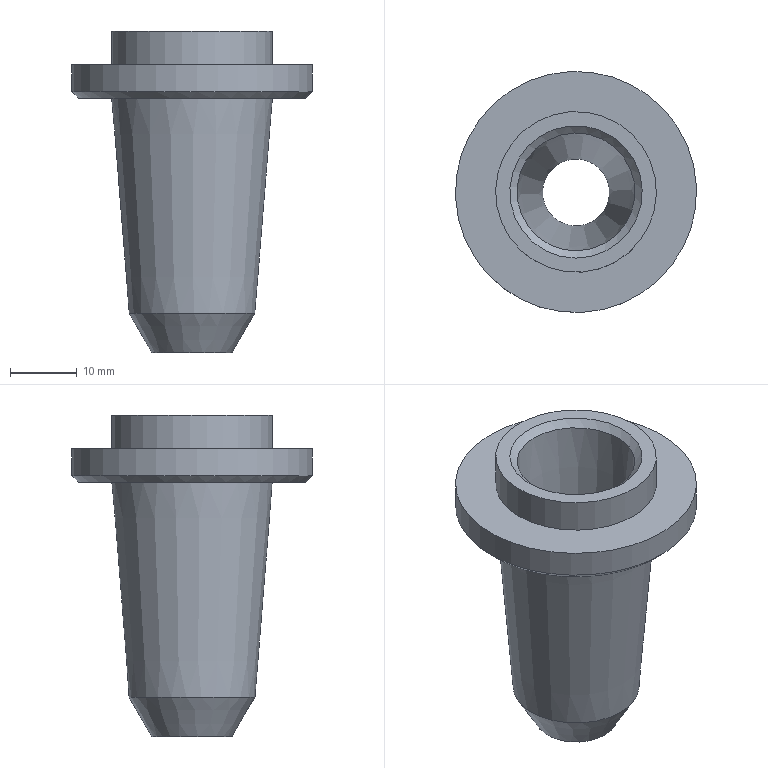Component | NX | LARGE_NOZZLE | 1 solid | 11 faces | box 36 x 36 x 48 mm | volume 12529 mm3 | cone 5 | plane 4 | cylinder 2 | commonest cylinder face diameters 24 x1 36 x1
STEP:
#1=CARTESIAN_POINT('',(0.,0.,0.));
#2=DIRECTION('',(0.,0.,1.));
#3=DIRECTION('',(1.,0.,0.));
#4=AXIS2_PLACEMENT_3D('',#1,#2,#3);
#5=CARTESIAN_POINT('',(1.601,2.184,25.889));
#6=VERTEX_POINT('',#5);
#7=CARTESIAN_POINT('',(10.284,5.784,25.889));
#8=DIRECTION('',(0.,0.,1.));
#9=DIRECTION('',(-0.9237,-0.383,0.));
#10=AXIS2_PLACEMENT_3D('',#7,#8,#9);
#11=CIRCLE('',#10,9.4);
#12=CARTESIAN_POINT('',(10.284,5.784,58.));
#13=DIRECTION('',(0.,0.,1.));
#14=DIRECTION('',(-0.9237,-0.383,0.));
#15=AXIS2_PLACEMENT_3D('',#12,#13,#14);
#16=CONICAL_SURFACE('',#15,12.,0.08079);
#17=CARTESIAN_POINT('',(0.,-32.111));
#18=DIRECTION('',(1.,0.));
#19=VECTOR('',#18,1.);
#20=LINE('',#17,#19);
#21=(GEOMETRIC_REPRESENTATION_CONTEXT(2)PARAMETRIC_REPRESENTATION_CONTEXT()REPRESENTATION_CONTEXT('',''));
#22=DEFINITIONAL_REPRESENTATION('',(#20),#21);
#23=PCURVE('',#16,#22);
#24=CARTESIAN_POINT('',(10.284,5.784,25.889));
#25=DIRECTION('',(0.,0.,1.));
#26=DIRECTION('',(-0.9237,-0.383,0.));
#27=AXIS2_PLACEMENT_3D('',#24,#25,#26);
#28=CONICAL_SURFACE('',#27,9.4,0.5236);
#29=CARTESIAN_POINT('',(0.,0.));
#30=DIRECTION('',(1.,0.));
#31=VECTOR('',#30,1.);
#32=LINE('',#29,#31);
#33=(GEOMETRIC_REPRESENTATION_CONTEXT(2)PARAMETRIC_REPRESENTATION_CONTEXT()REPRESENTATION_CONTEXT('',''));
#34=DEFINITIONAL_REPRESENTATION('',(#32),#33);
#35=PCURVE('',#28,#34);
#36=SURFACE_CURVE('',#11,(#23,#35),.PCURVE_S1.);
#37=EDGE_CURVE('',#6,#6,#36,.T.);
#38=ORIENTED_EDGE('',*,*,#37,.T.);
#39=CARTESIAN_POINT('',(-0.8005,1.188,58.));
#40=VERTEX_POINT('',#39);
#41=CARTESIAN_POINT('',(1.601,2.184,25.889));
#42=CARTESIAN_POINT('',(-0.8005,1.188,58.));
#43=B_SPLINE_CURVE_WITH_KNOTS('',1,(#41,#42),.UNSPECIFIED.,.F.,.F.,(2,2),(-32.216,0.),.PIECEWISE_BEZIER_KNOTS.);
#44=CARTESIAN_POINT('',(6.283,0.));
#45=DIRECTION('',(0.,1.));
#46=VECTOR('',#45,1.);
#47=LINE('',#44,#46);
#48=(GEOMETRIC_REPRESENTATION_CONTEXT(2)PARAMETRIC_REPRESENTATION_CONTEXT()REPRESENTATION_CONTEXT('',''));
#49=DEFINITIONAL_REPRESENTATION('',(#47),#48);
#50=PCURVE('',#16,#49);
#51=CARTESIAN_POINT('',(0.,0.));
#52=DIRECTION('',(0.,1.));
#53=VECTOR('',#52,1.);
#54=LINE('',#51,#53);
#55=(GEOMETRIC_REPRESENTATION_CONTEXT(2)PARAMETRIC_REPRESENTATION_CONTEXT()REPRESENTATION_CONTEXT('',''));
#56=DEFINITIONAL_REPRESENTATION('',(#54),#55);
#57=PCURVE('',#16,#56);
#58=SEAM_CURVE('',#43,(#50,#57),.PCURVE_S1.);
#59=EDGE_CURVE('',#6,#40,#58,.T.);
#60=ORIENTED_EDGE('',*,*,#59,.T.);
#61=CARTESIAN_POINT('',(10.284,5.784,58.));
#62=DIRECTION('',(0.,0.,1.));
#63=DIRECTION('',(-0.9237,-0.383,0.));
#64=AXIS2_PLACEMENT_3D('',#61,#62,#63);
#65=CIRCLE('',#64,12.);
#66=CARTESIAN_POINT('',(0.,0.));
#67=DIRECTION('',(1.,0.));
#68=VECTOR('',#67,1.);
#69=LINE('',#66,#68);
#70=(GEOMETRIC_REPRESENTATION_CONTEXT(2)PARAMETRIC_REPRESENTATION_CONTEXT()REPRESENTATION_CONTEXT('',''));
#71=DEFINITIONAL_REPRESENTATION('',(#69),#70);
#72=PCURVE('',#16,#71);
#73=CARTESIAN_POINT('',(17.179,-10.843,58.));
#74=DIRECTION('',(0.,0.,-1.));
#75=DIRECTION('',(0.9237,0.383,0.));
#76=AXIS2_PLACEMENT_3D('',#73,#74,#75);
#77=PLANE('',#76);
#78=CARTESIAN_POINT('',(-12.,-18.));
#79=CARTESIAN_POINT('',(-12.,2.785));
#80=CARTESIAN_POINT('',(6.,-7.608));
#81=CARTESIAN_POINT('',(24.,-18.));
#82=CARTESIAN_POINT('',(6.,-28.392));
#83=CARTESIAN_POINT('',(-12.,-38.785));
#84=CARTESIAN_POINT('',(-12.,-18.));
#85=(BOUNDED_CURVE()B_SPLINE_CURVE(2,(#78,#79,#80,#81,#82,#83,#84),.UNSPECIFIED.,.T.,.F.)B_SPLINE_CURVE_WITH_KNOTS((1,2,2,2,2,1),(-2.094,0.,2.094,4.189,6.283,8.378),.UNSPECIFIED.)CURVE()GEOMETRIC_REPRESENTATION_ITEM()RATIONAL_B_SPLINE_CURVE((1.,0.5,1.,0.5,1.,0.5,1.))REPRESENTATION_ITEM(''));
#86=(GEOMETRIC_REPRESENTATION_CONTEXT(2)PARAMETRIC_REPRESENTATION_CONTEXT()REPRESENTATION_CONTEXT('',''));
#87=DEFINITIONAL_REPRESENTATION('',(#85),#86);
#88=PCURVE('',#77,#87);
#89=SURFACE_CURVE('',#65,(#72,#88),.PCURVE_S1.);
#90=EDGE_CURVE('',#40,#40,#89,.T.);
#91=ORIENTED_EDGE('',*,*,#90,.F.);
#92=ORIENTED_EDGE('',*,*,#59,.F.);
#93=EDGE_LOOP('',(#38,#60,#91,#92));
#94=FACE_BOUND('',#93,.T.);
#95=ADVANCED_FACE('',(#94),#16,.T.);
#96=CARTESIAN_POINT('',(4.742,3.486,20.));
#97=VERTEX_POINT('',#96);
#98=CARTESIAN_POINT('',(10.284,5.784,20.));
#99=DIRECTION('',(0.,0.,1.));
#100=DIRECTION('',(-0.9237,-0.383,0.));
#101=AXIS2_PLACEMENT_3D('',#98,#99,#100);
#102=CIRCLE('',#101,6.);
#103=CARTESIAN_POINT('',(0.,-5.889));
#104=DIRECTION('',(1.,0.));
#105=VECTOR('',#104,1.);
#106=LINE('',#103,#105);
#107=(GEOMETRIC_REPRESENTATION_CONTEXT(2)PARAMETRIC_REPRESENTATION_CONTEXT()REPRESENTATION_CONTEXT('',''));
#108=DEFINITIONAL_REPRESENTATION('',(#106),#107);
#109=PCURVE('',#28,#108);
#110=CARTESIAN_POINT('',(12.583,0.2419,20.));
#111=DIRECTION('',(0.,0.,-1.));
#112=DIRECTION('',(0.9237,0.383,0.));
#113=AXIS2_PLACEMENT_3D('',#110,#111,#112);
#114=PLANE('',#113);
#115=CARTESIAN_POINT('',(-6.,-6.));
#116=CARTESIAN_POINT('',(-6.,4.392));
#117=CARTESIAN_POINT('',(3.,-0.8038));
#118=CARTESIAN_POINT('',(12.,-6.));
#119=CARTESIAN_POINT('',(3.,-11.196));
#120=CARTESIAN_POINT('',(-6.,-16.392));
#121=CARTESIAN_POINT('',(-6.,-6.));
#122=(BOUNDED_CURVE()B_SPLINE_CURVE(2,(#115,#116,#117,#118,#119,#120,#121),.UNSPECIFIED.,.T.,.F.)B_SPLINE_CURVE_WITH_KNOTS((1,2,2,2,2,1),(-2.094,0.,2.094,4.189,6.283,8.378),.UNSPECIFIED.)CURVE()GEOMETRIC_REPRESENTATION_ITEM()RATIONAL_B_SPLINE_CURVE((1.,0.5,1.,0.5,1.,0.5,1.))REPRESENTATION_ITEM(''));
#123=(GEOMETRIC_REPRESENTATION_CONTEXT(2)PARAMETRIC_REPRESENTATION_CONTEXT()REPRESENTATION_CONTEXT('',''));
#124=DEFINITIONAL_REPRESENTATION('',(#122),#123);
#125=PCURVE('',#114,#124);
#126=SURFACE_CURVE('',#102,(#109,#125),.PCURVE_S1.);
#127=EDGE_CURVE('',#97,#97,#126,.T.);
#128=ORIENTED_EDGE('',*,*,#127,.T.);
#129=CARTESIAN_POINT('',(4.742,3.486,20.));
#130=CARTESIAN_POINT('',(1.601,2.184,25.889));
#131=B_SPLINE_CURVE_WITH_KNOTS('',1,(#129,#130),.UNSPECIFIED.,.F.,.F.,(2,2),(-6.8,0.),.PIECEWISE_BEZIER_KNOTS.);
#132=CARTESIAN_POINT('',(6.283,0.));
#133=DIRECTION('',(0.,1.));
#134=VECTOR('',#133,1.);
#135=LINE('',#132,#134);
#136=(GEOMETRIC_REPRESENTATION_CONTEXT(2)PARAMETRIC_REPRESENTATION_CONTEXT()REPRESENTATION_CONTEXT('',''));
#137=DEFINITIONAL_REPRESENTATION('',(#135),#136);
#138=PCURVE('',#28,#137);
#139=CARTESIAN_POINT('',(0.,0.));
#140=DIRECTION('',(0.,1.));
#141=VECTOR('',#140,1.);
#142=LINE('',#139,#141);
#143=(GEOMETRIC_REPRESENTATION_CONTEXT(2)PARAMETRIC_REPRESENTATION_CONTEXT()REPRESENTATION_CONTEXT('',''));
#144=DEFINITIONAL_REPRESENTATION('',(#142),#143);
#145=PCURVE('',#28,#144);
#146=SEAM_CURVE('',#131,(#138,#145),.PCURVE_S1.);
#147=EDGE_CURVE('',#97,#6,#146,.T.);
#148=ORIENTED_EDGE('',*,*,#147,.T.);
#149=ORIENTED_EDGE('',*,*,#37,.F.);
#150=ORIENTED_EDGE('',*,*,#147,.F.);
#151=EDGE_LOOP('',(#128,#148,#149,#150));
#152=FACE_BOUND('',#151,.T.);
#153=ADVANCED_FACE('',(#152),#28,.T.);
#154=CARTESIAN_POINT('',(5.666,3.869,20.));
#155=VERTEX_POINT('',#154);
#156=CARTESIAN_POINT('',(10.284,5.784,20.));
#157=DIRECTION('',(0.,0.,1.));
#158=DIRECTION('',(-0.9237,-0.383,0.));
#159=AXIS2_PLACEMENT_3D('',#156,#157,#158);
#160=CIRCLE('',#159,5.);
#161=CARTESIAN_POINT('',(-5.,-6.));
#162=CARTESIAN_POINT('',(-5.,2.66));
#163=CARTESIAN_POINT('',(2.5,-1.67));
#164=CARTESIAN_POINT('',(10.,-6.));
#165=CARTESIAN_POINT('',(2.5,-10.33));
#166=CARTESIAN_POINT('',(-5.,-14.66));
#167=CARTESIAN_POINT('',(-5.,-6.));
#168=(BOUNDED_CURVE()B_SPLINE_CURVE(2,(#161,#162,#163,#164,#165,#166,#167),.UNSPECIFIED.,.T.,.F.)B_SPLINE_CURVE_WITH_KNOTS((1,2,2,2,2,1),(-2.094,0.,2.094,4.189,6.283,8.378),.UNSPECIFIED.)CURVE()GEOMETRIC_REPRESENTATION_ITEM()RATIONAL_B_SPLINE_CURVE((1.,0.5,1.,0.5,1.,0.5,1.))REPRESENTATION_ITEM(''));
#169=(GEOMETRIC_REPRESENTATION_CONTEXT(2)PARAMETRIC_REPRESENTATION_CONTEXT()REPRESENTATION_CONTEXT('',''));
#170=DEFINITIONAL_REPRESENTATION('',(#168),#169);
#171=PCURVE('',#114,#170);
#172=CARTESIAN_POINT('',(10.284,5.784,20.));
#173=DIRECTION('',(0.,0.,1.));
#174=DIRECTION('',(-0.9237,-0.383,0.));
#175=AXIS2_PLACEMENT_3D('',#172,#173,#174);
#176=CONICAL_SURFACE('',#175,5.,0.08079);
#177=CARTESIAN_POINT('',(0.,0.));
#178=DIRECTION('',(1.,0.));
#179=VECTOR('',#178,1.);
#180=LINE('',#177,#179);
#181=(GEOMETRIC_REPRESENTATION_CONTEXT(2)PARAMETRIC_REPRESENTATION_CONTEXT()REPRESENTATION_CONTEXT('',''));
#182=DEFINITIONAL_REPRESENTATION('',(#180),#181);
#183=PCURVE('',#176,#182);
#184=SURFACE_CURVE('',#160,(#171,#183),.PCURVE_S1.);
#185=EDGE_CURVE('',#155,#155,#184,.T.);
#186=ORIENTED_EDGE('',*,*,#185,.T.);
#187=EDGE_LOOP('',(#186));
#188=FACE_BOUND('',#187,.T.);
#189=ORIENTED_EDGE('',*,*,#127,.F.);
#190=EDGE_LOOP('',(#189));
#191=FACE_BOUND('',#190,.T.);
#192=ADVANCED_FACE('',(#188,#191),#114,.T.);
#193=CARTESIAN_POINT('',(2.15,2.411,67.003));
#194=VERTEX_POINT('',#193);
#195=CARTESIAN_POINT('',(18.418,9.157,67.003));
#196=VERTEX_POINT('',#195);
#197=CARTESIAN_POINT('',(10.284,5.784,67.003));
#198=DIRECTION('',(0.,0.,1.));
#199=DIRECTION('',(0.9237,0.383,0.));
#200=AXIS2_PLACEMENT_3D('',#197,#198,#199);
#201=CIRCLE('',#200,8.806);
#202=CARTESIAN_POINT('',(-3.142,47.003));
#203=DIRECTION('',(1.,0.));
#204=VECTOR('',#203,1.);
#205=LINE('',#202,#204);
#206=(GEOMETRIC_REPRESENTATION_CONTEXT(2)PARAMETRIC_REPRESENTATION_CONTEXT()REPRESENTATION_CONTEXT('',''));
#207=DEFINITIONAL_REPRESENTATION('',(#205),#206);
#208=PCURVE('',#176,#207);
#209=CARTESIAN_POINT('',(10.284,5.784,67.003));
#210=DIRECTION('',(0.,0.,1.));
#211=DIRECTION('',(-0.9237,-0.383,0.));
#212=AXIS2_PLACEMENT_3D('',#209,#210,#211);
#213=CONICAL_SURFACE('',#212,8.806,0.8258);
#214=CARTESIAN_POINT('',(-3.142,0.));
#215=DIRECTION('',(1.,0.));
#216=VECTOR('',#215,1.);
#217=LINE('',#214,#216);
#218=(GEOMETRIC_REPRESENTATION_CONTEXT(2)PARAMETRIC_REPRESENTATION_CONTEXT()REPRESENTATION_CONTEXT('',''));
#219=DEFINITIONAL_REPRESENTATION('',(#217),#218);
#220=PCURVE('',#213,#219);
#221=SURFACE_CURVE('',#201,(#208,#220),.PCURVE_S1.);
#222=EDGE_CURVE('',#194,#196,#221,.T.);
#223=ORIENTED_EDGE('',*,*,#222,.F.);
#224=CARTESIAN_POINT('',(5.666,3.869,20.));
#225=CARTESIAN_POINT('',(2.15,2.411,67.003));
#226=B_SPLINE_CURVE_WITH_KNOTS('',1,(#224,#225),.UNSPECIFIED.,.F.,.F.,(2,2),(0.,47.157),.PIECEWISE_BEZIER_KNOTS.);
#227=CARTESIAN_POINT('',(0.,0.));
#228=DIRECTION('',(0.,1.));
#229=VECTOR('',#228,1.);
#230=LINE('',#227,#229);
#231=(GEOMETRIC_REPRESENTATION_CONTEXT(2)PARAMETRIC_REPRESENTATION_CONTEXT()REPRESENTATION_CONTEXT('',''));
#232=DEFINITIONAL_REPRESENTATION('',(#230),#231);
#233=PCURVE('',#176,#232);
#234=CARTESIAN_POINT('',(6.283,0.));
#235=DIRECTION('',(0.,1.));
#236=VECTOR('',#235,1.);
#237=LINE('',#234,#236);
#238=(GEOMETRIC_REPRESENTATION_CONTEXT(2)PARAMETRIC_REPRESENTATION_CONTEXT()REPRESENTATION_CONTEXT('',''));
#239=DEFINITIONAL_REPRESENTATION('',(#237),#238);
#240=PCURVE('',#176,#239);
#241=SEAM_CURVE('',#226,(#233,#240),.PCURVE_S1.);
#242=EDGE_CURVE('',#155,#194,#241,.T.);
#243=ORIENTED_EDGE('',*,*,#242,.F.);
#244=ORIENTED_EDGE('',*,*,#185,.T.);
#245=ORIENTED_EDGE('',*,*,#242,.T.);
#246=CARTESIAN_POINT('',(10.284,5.784,67.003));
#247=DIRECTION('',(0.,0.,1.));
#248=DIRECTION('',(0.9237,0.383,0.));
#249=AXIS2_PLACEMENT_3D('',#246,#247,#248);
#250=CIRCLE('',#249,8.806);
#251=CARTESIAN_POINT('',(3.142,47.003));
#252=DIRECTION('',(1.,0.));
#253=VECTOR('',#252,1.);
#254=LINE('',#251,#253);
#255=(GEOMETRIC_REPRESENTATION_CONTEXT(2)PARAMETRIC_REPRESENTATION_CONTEXT()REPRESENTATION_CONTEXT('',''));
#256=DEFINITIONAL_REPRESENTATION('',(#254),#255);
#257=PCURVE('',#176,#256);
#258=CARTESIAN_POINT('',(3.142,0.));
#259=DIRECTION('',(1.,-0.));
#260=VECTOR('',#259,1.);
#261=LINE('',#258,#260);
#262=(GEOMETRIC_REPRESENTATION_CONTEXT(2)PARAMETRIC_REPRESENTATION_CONTEXT()REPRESENTATION_CONTEXT('',''));
#263=DEFINITIONAL_REPRESENTATION('',(#261),#262);
#264=PCURVE('',#213,#263);
#265=SURFACE_CURVE('',#250,(#257,#264),.PCURVE_S1.);
#266=EDGE_CURVE('',#196,#194,#265,.T.);
#267=ORIENTED_EDGE('',*,*,#266,.F.);
#268=EDGE_LOOP('',(#223,#243,#244,#245,#267));
#269=FACE_BOUND('',#268,.F.);
#270=ADVANCED_FACE('',(#269),#176,.F.);
#271=CARTESIAN_POINT('',(1.152,1.997,68.));
#272=VERTEX_POINT('',#271);
#273=CARTESIAN_POINT('',(10.284,5.784,68.));
#274=DIRECTION('',(0.,0.,-1.));
#275=DIRECTION('',(-0.9237,-0.383,0.));
#276=AXIS2_PLACEMENT_3D('',#273,#274,#275);
#277=CIRCLE('',#276,9.887);
#278=CARTESIAN_POINT('',(13.688,-2.424,68.));
#279=DIRECTION('',(0.,0.,1.));
#280=DIRECTION('',(-0.9237,-0.383,0.));
#281=AXIS2_PLACEMENT_3D('',#278,#279,#280);
#282=PLANE('',#281);
#283=CARTESIAN_POINT('',(9.887,-8.887));
#284=CARTESIAN_POINT('',(9.887,-26.01));
#285=CARTESIAN_POINT('',(-4.943,-17.448));
#286=CARTESIAN_POINT('',(-19.773,-8.887));
#287=CARTESIAN_POINT('',(-4.943,-0.3245));
#288=CARTESIAN_POINT('',(9.887,8.237));
#289=CARTESIAN_POINT('',(9.887,-8.887));
#290=(BOUNDED_CURVE()B_SPLINE_CURVE(2,(#283,#284,#285,#286,#287,#288,#289),.UNSPECIFIED.,.T.,.F.)B_SPLINE_CURVE_WITH_KNOTS((1,2,2,2,2,1),(-2.094,0.,2.094,4.189,6.283,8.378),.UNSPECIFIED.)CURVE()GEOMETRIC_REPRESENTATION_ITEM()RATIONAL_B_SPLINE_CURVE((1.,0.5,1.,0.5,1.,0.5,1.))REPRESENTATION_ITEM(''));
#291=(GEOMETRIC_REPRESENTATION_CONTEXT(2)PARAMETRIC_REPRESENTATION_CONTEXT()REPRESENTATION_CONTEXT('',''));
#292=DEFINITIONAL_REPRESENTATION('',(#290),#291);
#293=PCURVE('',#282,#292);
#294=CARTESIAN_POINT('',(6.283,0.9967));
#295=DIRECTION('',(-1.,0.));
#296=VECTOR('',#295,1.);
#297=LINE('',#294,#296);
#298=(GEOMETRIC_REPRESENTATION_CONTEXT(2)PARAMETRIC_REPRESENTATION_CONTEXT()REPRESENTATION_CONTEXT('',''));
#299=DEFINITIONAL_REPRESENTATION('',(#297),#298);
#300=PCURVE('',#213,#299);
#301=SURFACE_CURVE('',#277,(#293,#300),.PCURVE_S1.);
#302=EDGE_CURVE('',#272,#272,#301,.T.);
#303=ORIENTED_EDGE('',*,*,#302,.T.);
#304=EDGE_LOOP('',(#303));
#305=FACE_BOUND('',#304,.T.);
#306=CARTESIAN_POINT('',(-0.8005,1.188,68.));
#307=VERTEX_POINT('',#306);
#308=CARTESIAN_POINT('',(10.284,5.784,68.));
#309=DIRECTION('',(0.,0.,1.));
#310=DIRECTION('',(-0.9237,-0.383,0.));
#311=AXIS2_PLACEMENT_3D('',#308,#309,#310);
#312=CIRCLE('',#311,12.);
#313=CARTESIAN_POINT('',(0.,-8.887));
#314=DIRECTION('',(1.,0.));
#315=AXIS2_PLACEMENT_2D('',#313,#314);
#316=CIRCLE('',#315,12.);
#317=(GEOMETRIC_REPRESENTATION_CONTEXT(2)PARAMETRIC_REPRESENTATION_CONTEXT()REPRESENTATION_CONTEXT('',''));
#318=DEFINITIONAL_REPRESENTATION('',(#316),#317);
#319=PCURVE('',#282,#318);
#320=CARTESIAN_POINT('',(10.284,5.784,68.));
#321=DIRECTION('',(0.,0.,1.));
#322=DIRECTION('',(-0.9237,-0.383,0.));
#323=AXIS2_PLACEMENT_3D('',#320,#321,#322);
#324=CYLINDRICAL_SURFACE('',#323,12.);
#325=CARTESIAN_POINT('',(0.,0.));
#326=DIRECTION('',(1.,0.));
#327=VECTOR('',#326,1.);
#328=LINE('',#325,#327);
#329=(GEOMETRIC_REPRESENTATION_CONTEXT(2)PARAMETRIC_REPRESENTATION_CONTEXT()REPRESENTATION_CONTEXT('',''));
#330=DEFINITIONAL_REPRESENTATION('',(#328),#329);
#331=PCURVE('',#324,#330);
#332=SURFACE_CURVE('',#312,(#319,#331),.PCURVE_S1.);
#333=EDGE_CURVE('',#307,#307,#332,.T.);
#334=ORIENTED_EDGE('',*,*,#333,.T.);
#335=EDGE_LOOP('',(#334));
#336=FACE_BOUND('',#335,.T.);
#337=ADVANCED_FACE('',(#305,#336),#282,.T.);
#338=CARTESIAN_POINT('',(-0.8005,1.188,63.));
#339=VERTEX_POINT('',#338);
#340=CARTESIAN_POINT('',(10.284,5.784,63.));
#341=DIRECTION('',(0.,0.,1.));
#342=DIRECTION('',(-0.9237,-0.383,0.));
#343=AXIS2_PLACEMENT_3D('',#340,#341,#342);
#344=CIRCLE('',#343,12.);
#345=CARTESIAN_POINT('',(0.,-5.));
#346=DIRECTION('',(1.,0.));
#347=VECTOR('',#346,1.);
#348=LINE('',#345,#347);
#349=(GEOMETRIC_REPRESENTATION_CONTEXT(2)PARAMETRIC_REPRESENTATION_CONTEXT()REPRESENTATION_CONTEXT('',''));
#350=DEFINITIONAL_REPRESENTATION('',(#348),#349);
#351=PCURVE('',#324,#350);
#352=CARTESIAN_POINT('',(14.881,-5.3,63.));
#353=DIRECTION('',(0.,0.,1.));
#354=DIRECTION('',(-0.9237,-0.383,0.));
#355=AXIS2_PLACEMENT_3D('',#352,#353,#354);
#356=PLANE('',#355);
#357=CARTESIAN_POINT('',(0.,-12.));
#358=DIRECTION('',(1.,0.));
#359=AXIS2_PLACEMENT_2D('',#357,#358);
#360=CIRCLE('',#359,12.);
#361=(GEOMETRIC_REPRESENTATION_CONTEXT(2)PARAMETRIC_REPRESENTATION_CONTEXT()REPRESENTATION_CONTEXT('',''));
#362=DEFINITIONAL_REPRESENTATION('',(#360),#361);
#363=PCURVE('',#356,#362);
#364=SURFACE_CURVE('',#344,(#351,#363),.PCURVE_S1.);
#365=EDGE_CURVE('',#339,#339,#364,.T.);
#366=ORIENTED_EDGE('',*,*,#365,.T.);
#367=CARTESIAN_POINT('',(-0.8005,1.188,63.));
#368=CARTESIAN_POINT('',(-0.8005,1.188,68.));
#369=B_SPLINE_CURVE_WITH_KNOTS('',1,(#367,#368),.UNSPECIFIED.,.F.,.F.,(2,2),(-5.,0.),.PIECEWISE_BEZIER_KNOTS.);
#370=CARTESIAN_POINT('',(6.283,0.));
#371=DIRECTION('',(0.,1.));
#372=VECTOR('',#371,1.);
#373=LINE('',#370,#372);
#374=(GEOMETRIC_REPRESENTATION_CONTEXT(2)PARAMETRIC_REPRESENTATION_CONTEXT()REPRESENTATION_CONTEXT('',''));
#375=DEFINITIONAL_REPRESENTATION('',(#373),#374);
#376=PCURVE('',#324,#375);
#377=CARTESIAN_POINT('',(0.,0.));
#378=DIRECTION('',(0.,1.));
#379=VECTOR('',#378,1.);
#380=LINE('',#377,#379);
#381=(GEOMETRIC_REPRESENTATION_CONTEXT(2)PARAMETRIC_REPRESENTATION_CONTEXT()REPRESENTATION_CONTEXT('',''));
#382=DEFINITIONAL_REPRESENTATION('',(#380),#381);
#383=PCURVE('',#324,#382);
#384=SEAM_CURVE('',#369,(#376,#383),.PCURVE_S1.);
#385=EDGE_CURVE('',#339,#307,#384,.T.);
#386=ORIENTED_EDGE('',*,*,#385,.T.);
#387=ORIENTED_EDGE('',*,*,#333,.F.);
#388=ORIENTED_EDGE('',*,*,#385,.F.);
#389=EDGE_LOOP('',(#366,#386,#387,#388));
#390=FACE_BOUND('',#389,.T.);
#391=ADVANCED_FACE('',(#390),#324,.T.);
#392=CARTESIAN_POINT('',(-6.343,-1.111,63.));
#393=VERTEX_POINT('',#392);
#394=CARTESIAN_POINT('',(10.284,5.784,63.));
#395=DIRECTION('',(0.,0.,1.));
#396=DIRECTION('',(-0.9237,-0.383,0.));
#397=AXIS2_PLACEMENT_3D('',#394,#395,#396);
#398=CIRCLE('',#397,18.);
#399=CARTESIAN_POINT('',(0.,-12.));
#400=DIRECTION('',(1.,0.));
#401=AXIS2_PLACEMENT_2D('',#399,#400);
#402=CIRCLE('',#401,18.);
#403=(GEOMETRIC_REPRESENTATION_CONTEXT(2)PARAMETRIC_REPRESENTATION_CONTEXT()REPRESENTATION_CONTEXT('',''));
#404=DEFINITIONAL_REPRESENTATION('',(#402),#403);
#405=PCURVE('',#356,#404);
#406=CARTESIAN_POINT('',(10.284,5.784,68.));
#407=DIRECTION('',(0.,0.,1.));
#408=DIRECTION('',(-0.9237,-0.383,0.));
#409=AXIS2_PLACEMENT_3D('',#406,#407,#408);
#410=CYLINDRICAL_SURFACE('',#409,18.);
#411=CARTESIAN_POINT('',(0.,-5.));
#412=DIRECTION('',(1.,0.));
#413=VECTOR('',#412,1.);
#414=LINE('',#411,#413);
#415=(GEOMETRIC_REPRESENTATION_CONTEXT(2)PARAMETRIC_REPRESENTATION_CONTEXT()REPRESENTATION_CONTEXT('',''));
#416=DEFINITIONAL_REPRESENTATION('',(#414),#415);
#417=PCURVE('',#410,#416);
#418=SURFACE_CURVE('',#398,(#405,#417),.PCURVE_S1.);
#419=EDGE_CURVE('',#393,#393,#418,.T.);
#420=ORIENTED_EDGE('',*,*,#419,.T.);
#421=EDGE_LOOP('',(#420));
#422=FACE_BOUND('',#421,.T.);
#423=ORIENTED_EDGE('',*,*,#365,.F.);
#424=EDGE_LOOP('',(#423));
#425=FACE_BOUND('',#424,.T.);
#426=ADVANCED_FACE('',(#422,#425),#356,.T.);
#427=CARTESIAN_POINT('',(26.911,12.679,59.));
#428=VERTEX_POINT('',#427);
#429=CARTESIAN_POINT('',(-6.343,-1.111,59.));
#430=VERTEX_POINT('',#429);
#431=CARTESIAN_POINT('',(10.284,5.784,59.));
#432=DIRECTION('',(0.,0.,1.));
#433=DIRECTION('',(0.9237,0.383,0.));
#434=AXIS2_PLACEMENT_3D('',#431,#432,#433);
#435=CIRCLE('',#434,18.);
#436=CARTESIAN_POINT('',(3.142,-9.));
#437=DIRECTION('',(1.,0.));
#438=VECTOR('',#437,1.);
#439=LINE('',#436,#438);
#440=(GEOMETRIC_REPRESENTATION_CONTEXT(2)PARAMETRIC_REPRESENTATION_CONTEXT()REPRESENTATION_CONTEXT('',''));
#441=DEFINITIONAL_REPRESENTATION('',(#439),#440);
#442=PCURVE('',#410,#441);
#443=CARTESIAN_POINT('',(10.284,5.784,59.));
#444=DIRECTION('',(0.,0.,1.));
#445=DIRECTION('',(-0.9237,-0.383,0.));
#446=AXIS2_PLACEMENT_3D('',#443,#444,#445);
#447=CONICAL_SURFACE('',#446,18.,0.7854);
#448=CARTESIAN_POINT('',(3.142,0.));
#449=DIRECTION('',(1.,0.));
#450=VECTOR('',#449,1.);
#451=LINE('',#448,#450);
#452=(GEOMETRIC_REPRESENTATION_CONTEXT(2)PARAMETRIC_REPRESENTATION_CONTEXT()REPRESENTATION_CONTEXT('',''));
#453=DEFINITIONAL_REPRESENTATION('',(#451),#452);
#454=PCURVE('',#447,#453);
#455=SURFACE_CURVE('',#435,(#442,#454),.PCURVE_S1.);
#456=EDGE_CURVE('',#428,#430,#455,.T.);
#457=ORIENTED_EDGE('',*,*,#456,.T.);
#458=CARTESIAN_POINT('',(-6.343,-1.111,59.));
#459=CARTESIAN_POINT('',(-6.343,-1.111,63.));
#460=B_SPLINE_CURVE_WITH_KNOTS('',1,(#458,#459),.UNSPECIFIED.,.F.,.F.,(2,2),(-9.,-5.),.PIECEWISE_BEZIER_KNOTS.);
#461=CARTESIAN_POINT('',(6.283,0.));
#462=DIRECTION('',(0.,1.));
#463=VECTOR('',#462,1.);
#464=LINE('',#461,#463);
#465=(GEOMETRIC_REPRESENTATION_CONTEXT(2)PARAMETRIC_REPRESENTATION_CONTEXT()REPRESENTATION_CONTEXT('',''));
#466=DEFINITIONAL_REPRESENTATION('',(#464),#465);
#467=PCURVE('',#410,#466);
#468=CARTESIAN_POINT('',(0.,0.));
#469=DIRECTION('',(0.,1.));
#470=VECTOR('',#469,1.);
#471=LINE('',#468,#470);
#472=(GEOMETRIC_REPRESENTATION_CONTEXT(2)PARAMETRIC_REPRESENTATION_CONTEXT()REPRESENTATION_CONTEXT('',''));
#473=DEFINITIONAL_REPRESENTATION('',(#471),#472);
#474=PCURVE('',#410,#473);
#475=SEAM_CURVE('',#460,(#467,#474),.PCURVE_S1.);
#476=EDGE_CURVE('',#430,#393,#475,.T.);
#477=ORIENTED_EDGE('',*,*,#476,.T.);
#478=ORIENTED_EDGE('',*,*,#419,.F.);
#479=ORIENTED_EDGE('',*,*,#476,.F.);
#480=CARTESIAN_POINT('',(10.284,5.784,59.));
#481=DIRECTION('',(0.,0.,1.));
#482=DIRECTION('',(0.9237,0.383,0.));
#483=AXIS2_PLACEMENT_3D('',#480,#481,#482);
#484=CIRCLE('',#483,18.);
#485=CARTESIAN_POINT('',(-3.142,-9.));
#486=DIRECTION('',(1.,0.));
#487=VECTOR('',#486,1.);
#488=LINE('',#485,#487);
#489=(GEOMETRIC_REPRESENTATION_CONTEXT(2)PARAMETRIC_REPRESENTATION_CONTEXT()REPRESENTATION_CONTEXT('',''));
#490=DEFINITIONAL_REPRESENTATION('',(#488),#489);
#491=PCURVE('',#410,#490);
#492=CARTESIAN_POINT('',(3.142,0.));
#493=DIRECTION('',(1.,0.));
#494=VECTOR('',#493,1.);
#495=LINE('',#492,#494);
#496=(GEOMETRIC_REPRESENTATION_CONTEXT(2)PARAMETRIC_REPRESENTATION_CONTEXT()REPRESENTATION_CONTEXT('',''));
#497=DEFINITIONAL_REPRESENTATION('',(#495),#496);
#498=PCURVE('',#447,#497);
#499=SURFACE_CURVE('',#484,(#491,#498),.PCURVE_S1.);
#500=EDGE_CURVE('',#430,#428,#499,.T.);
#501=ORIENTED_EDGE('',*,*,#500,.T.);
#502=EDGE_LOOP('',(#457,#477,#478,#479,#501));
#503=FACE_BOUND('',#502,.T.);
#504=ADVANCED_FACE('',(#503),#410,.T.);
#505=CARTESIAN_POINT('',(25.988,12.296,58.));
#506=VERTEX_POINT('',#505);
#507=CARTESIAN_POINT('',(10.284,5.784,58.));
#508=DIRECTION('',(0.,0.,-1.));
#509=DIRECTION('',(0.9237,0.383,0.));
#510=AXIS2_PLACEMENT_3D('',#507,#508,#509);
#511=CIRCLE('',#510,17.);
#512=CARTESIAN_POINT('',(-0.,-18.));
#513=DIRECTION('',(1.,0.));
#514=AXIS2_PLACEMENT_2D('',#512,#513);
#515=CIRCLE('',#514,17.);
#516=(GEOMETRIC_REPRESENTATION_CONTEXT(2)PARAMETRIC_REPRESENTATION_CONTEXT()REPRESENTATION_CONTEXT('',''));
#517=DEFINITIONAL_REPRESENTATION('',(#515),#516);
#518=PCURVE('',#77,#517);
#519=CARTESIAN_POINT('',(9.425,-1.));
#520=DIRECTION('',(-1.,-0.));
#521=VECTOR('',#520,1.);
#522=LINE('',#519,#521);
#523=(GEOMETRIC_REPRESENTATION_CONTEXT(2)PARAMETRIC_REPRESENTATION_CONTEXT()REPRESENTATION_CONTEXT('',''));
#524=DEFINITIONAL_REPRESENTATION('',(#522),#523);
#525=PCURVE('',#447,#524);
#526=SURFACE_CURVE('',#511,(#518,#525),.PCURVE_S1.);
#527=EDGE_CURVE('',#506,#506,#526,.T.);
#528=ORIENTED_EDGE('',*,*,#527,.T.);
#529=EDGE_LOOP('',(#528));
#530=FACE_BOUND('',#529,.T.);
#531=ORIENTED_EDGE('',*,*,#90,.T.);
#532=EDGE_LOOP('',(#531));
#533=FACE_BOUND('',#532,.T.);
#534=ADVANCED_FACE('',(#530,#533),#77,.T.);
#535=ORIENTED_EDGE('',*,*,#302,.T.);
#536=CARTESIAN_POINT('',(2.15,2.411,67.003));
#537=CARTESIAN_POINT('',(1.152,1.997,68.));
#538=B_SPLINE_CURVE_WITH_KNOTS('',1,(#536,#537),.UNSPECIFIED.,.F.,.F.,(2,2),(0.,1.47),.PIECEWISE_BEZIER_KNOTS.);
#539=CARTESIAN_POINT('',(0.,0.));
#540=DIRECTION('',(0.,1.));
#541=VECTOR('',#540,1.);
#542=LINE('',#539,#541);
#543=(GEOMETRIC_REPRESENTATION_CONTEXT(2)PARAMETRIC_REPRESENTATION_CONTEXT()REPRESENTATION_CONTEXT('',''));
#544=DEFINITIONAL_REPRESENTATION('',(#542),#543);
#545=PCURVE('',#213,#544);
#546=CARTESIAN_POINT('',(6.283,0.));
#547=DIRECTION('',(0.,1.));
#548=VECTOR('',#547,1.);
#549=LINE('',#546,#548);
#550=(GEOMETRIC_REPRESENTATION_CONTEXT(2)PARAMETRIC_REPRESENTATION_CONTEXT()REPRESENTATION_CONTEXT('',''));
#551=DEFINITIONAL_REPRESENTATION('',(#549),#550);
#552=PCURVE('',#213,#551);
#553=SEAM_CURVE('',#538,(#545,#552),.PCURVE_S1.);
#554=EDGE_CURVE('',#194,#272,#553,.T.);
#555=ORIENTED_EDGE('',*,*,#554,.F.);
#556=ORIENTED_EDGE('',*,*,#222,.T.);
#557=ORIENTED_EDGE('',*,*,#266,.T.);
#558=ORIENTED_EDGE('',*,*,#554,.T.);
#559=EDGE_LOOP('',(#535,#555,#556,#557,#558));
#560=FACE_BOUND('',#559,.F.);
#561=ADVANCED_FACE('',(#560),#213,.F.);
#562=ORIENTED_EDGE('',*,*,#527,.F.);
#563=CARTESIAN_POINT('',(25.988,12.296,58.));
#564=CARTESIAN_POINT('',(26.911,12.679,59.));
#565=B_SPLINE_CURVE_WITH_KNOTS('',1,(#563,#564),.UNSPECIFIED.,.F.,.F.,(2,2),(-1.414,0.),.PIECEWISE_BEZIER_KNOTS.);
#566=CARTESIAN_POINT('',(9.425,0.));
#567=DIRECTION('',(0.,1.));
#568=VECTOR('',#567,1.);
#569=LINE('',#566,#568);
#570=(GEOMETRIC_REPRESENTATION_CONTEXT(2)PARAMETRIC_REPRESENTATION_CONTEXT()REPRESENTATION_CONTEXT('',''));
#571=DEFINITIONAL_REPRESENTATION('',(#569),#570);
#572=PCURVE('',#447,#571);
#573=CARTESIAN_POINT('',(3.142,0.));
#574=DIRECTION('',(0.,1.));
#575=VECTOR('',#574,1.);
#576=LINE('',#573,#575);
#577=(GEOMETRIC_REPRESENTATION_CONTEXT(2)PARAMETRIC_REPRESENTATION_CONTEXT()REPRESENTATION_CONTEXT('',''));
#578=DEFINITIONAL_REPRESENTATION('',(#576),#577);
#579=PCURVE('',#447,#578);
#580=SEAM_CURVE('',#565,(#572,#579),.PCURVE_S1.);
#581=EDGE_CURVE('',#506,#428,#580,.T.);
#582=ORIENTED_EDGE('',*,*,#581,.T.);
#583=ORIENTED_EDGE('',*,*,#500,.F.);
#584=ORIENTED_EDGE('',*,*,#456,.F.);
#585=ORIENTED_EDGE('',*,*,#581,.F.);
#586=EDGE_LOOP('',(#562,#582,#583,#584,#585));
#587=FACE_BOUND('',#586,.T.);
#588=ADVANCED_FACE('',(#587),#447,.T.);
#589=CLOSED_SHELL('',(#95,#153,#192,#270,#337,#391,#426,#504,#534,#561,#588));
#590=MANIFOLD_SOLID_BREP('',#589);
#591=(LENGTH_UNIT()NAMED_UNIT(*)SI_UNIT(.MILLI.,.METRE.));
#592=UNCERTAINTY_MEASURE_WITH_UNIT(LENGTH_MEASURE(0.00001),#591,'','');
#593=(NAMED_UNIT(*)PLANE_ANGLE_UNIT()SI_UNIT($,.RADIAN.));
#594=(NAMED_UNIT(*)SI_UNIT($,.STERADIAN.)SOLID_ANGLE_UNIT());
#595=(GEOMETRIC_REPRESENTATION_CONTEXT(3)GLOBAL_UNCERTAINTY_ASSIGNED_CONTEXT((#592))GLOBAL_UNIT_ASSIGNED_CONTEXT((#591,#593,#594))REPRESENTATION_CONTEXT('',''));
#596=ADVANCED_BREP_SHAPE_REPRESENTATION('',(#4,#590),#595);